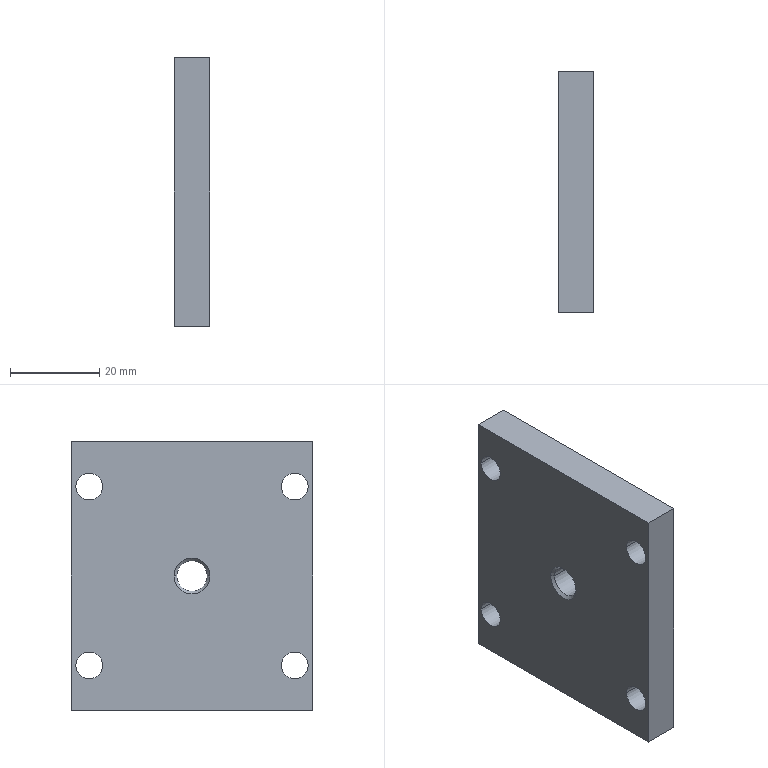Component | SolidWorks | Cover-1 | 1 solid | 18 faces | box 8 x 54 x 60 mm | volume 24720 mm3 | cylinder 10 | plane 6 | cone 2 | commonest cylinder face diameters 6 x8 6.8 x2
build123d program:
from build123d import *

# Parameters (mm, degrees)
SKETCH1_W                                            = 54
SKETCH1_H                                            = 60
BOSS_EXTRUDE1_DEPTH                                  = 8
F_6_0_6_DIAMETER_HOLE1_D                             = 6
TAPERED_COUNTERSUNK_HOLE1_FOR_M6_FLAT_HE_D           = 6.8
TAPERED_COUNTERSUNK_HOLE1_FOR_M6_FLAT_HE_CSINK_D     = 8.05
TAPERED_COUNTERSUNK_HOLE1_FOR_M6_FLAT_HE_CSINK_ANGLE = 90


with BuildPart() as part:
    # Sketch1 → Boss-Extrude1 (new body)
    with BuildSketch(Plane.XY.offset(4)):
        Rectangle(SKETCH1_W, SKETCH1_H)
    extrude(amount=-BOSS_EXTRUDE1_DEPTH)

    # 6.0 _6_ Diameter Hole1 (through all)
    with Locations(Plane(origin=(0, 0, -4), x_dir=(-1, 0, 0), z_dir=(0, 0, -1))):
        with Locations((-23, -20), (23, -20), (23, 20), (-23, 20)):
            Hole(F_6_0_6_DIAMETER_HOLE1_D / 2)

    # Tapered Countersunk Hole1 for M6 Flat He (through all)
    with Locations(Plane.XY.offset(4)):
        with Locations((0, 0)):
            CounterSinkHole(TAPERED_COUNTERSUNK_HOLE1_FOR_M6_FLAT_HE_D / 2, TAPERED_COUNTERSUNK_HOLE1_FOR_M6_FLAT_HE_CSINK_D / 2, counter_sink_angle=TAPERED_COUNTERSUNK_HOLE1_FOR_M6_FLAT_HE_CSINK_ANGLE)


solid = part.part

# Placed as in the assembly
solid = solid.moved(Location((-417, 405.75, -73.487), (90, -90, 0)))
STEP:
#1=COLOUR_RGB('',0.7922,0.8196,0.9333);
#2=FILL_AREA_STYLE_COLOUR('',#1);
#3=FILL_AREA_STYLE('',(#2));
#4=SURFACE_STYLE_FILL_AREA(#3);
#5=SURFACE_SIDE_STYLE('',(#4));
#6=SURFACE_STYLE_USAGE(.BOTH.,#5);
#7=PRESENTATION_STYLE_ASSIGNMENT((#6));
#8=CARTESIAN_POINT('',(-16.55,16.108,-2.893));
#9=VERTEX_POINT('',#8);
#10=CARTESIAN_POINT('',(-16.55,15.841,-2.893));
#11=VERTEX_POINT('',#10);
#12=CARTESIAN_POINT('',(-16.55,15.974,-2.893));
#13=DIRECTION('',(-1.,0.,-0.));
#14=DIRECTION('',(0.,-1.,0.));
#15=AXIS2_PLACEMENT_3D('',#12,#13,#14);
#16=CIRCLE('',#15,0.1339);
#17=EDGE_CURVE('',#9,#11,#16,.T.);
#18=ORIENTED_EDGE('',*,*,#17,.F.);
#19=CARTESIAN_POINT('',(-16.575,16.133,-2.893));
#20=VERTEX_POINT('',#19);
#21=CARTESIAN_POINT('',(-16.575,16.133,-2.893));
#22=DIRECTION('',(-0.7071,0.7071,0.));
#23=VECTOR('',#22,39.37);
#24=LINE('',#21,#23);
#25=EDGE_CURVE('',#9,#20,#24,.T.);
#26=ORIENTED_EDGE('',*,*,#25,.T.);
#27=CARTESIAN_POINT('',(-16.575,15.816,-2.893));
#28=VERTEX_POINT('',#27);
#29=CARTESIAN_POINT('',(-16.575,15.974,-2.893));
#30=DIRECTION('',(-1.,0.,-0.));
#31=DIRECTION('',(0.,-1.,0.));
#32=AXIS2_PLACEMENT_3D('',#29,#30,#31);
#33=CIRCLE('',#32,0.1585);
#34=EDGE_CURVE('',#20,#28,#33,.T.);
#35=ORIENTED_EDGE('',*,*,#34,.T.);
#36=CARTESIAN_POINT('',(-16.575,15.816,-2.893));
#37=DIRECTION('',(-0.7071,-0.7071,-0.));
#38=VECTOR('',#37,39.37);
#39=LINE('',#36,#38);
#40=EDGE_CURVE('',#11,#28,#39,.T.);
#41=ORIENTED_EDGE('',*,*,#40,.F.);
#42=EDGE_LOOP('',(#18,#26,#35,#41));
#43=FACE_OUTER_BOUND('',#42,.T.);
#44=CARTESIAN_POINT('',(-16.575,15.974,-2.893));
#45=DIRECTION('',(-1.,0.,-0.));
#46=DIRECTION('',(0.,-1.,0.));
#47=AXIS2_PLACEMENT_3D('',#44,#45,#46);
#48=CONICAL_SURFACE('',#47,0.1585,0.7854);
#49=ADVANCED_FACE('',(#43),#48,.F.);
#50=CARTESIAN_POINT('',(-16.26,16.108,-2.893));
#51=VERTEX_POINT('',#50);
#52=CARTESIAN_POINT('',(-16.26,15.841,-2.893));
#53=VERTEX_POINT('',#52);
#54=CARTESIAN_POINT('',(-16.26,15.974,-2.893));
#55=DIRECTION('',(-1.,0.,-0.));
#56=DIRECTION('',(0.,-1.,0.));
#57=AXIS2_PLACEMENT_3D('',#54,#55,#56);
#58=CIRCLE('',#57,0.1339);
#59=EDGE_CURVE('',#51,#53,#58,.T.);
#60=ORIENTED_EDGE('',*,*,#59,.F.);
#61=CARTESIAN_POINT('',(-16.575,16.108,-2.893));
#62=DIRECTION('',(-1.,0.,-0.));
#63=VECTOR('',#62,39.37);
#64=LINE('',#61,#63);
#65=EDGE_CURVE('',#51,#9,#64,.T.);
#66=ORIENTED_EDGE('',*,*,#65,.T.);
#67=ORIENTED_EDGE('',*,*,#17,.T.);
#68=CARTESIAN_POINT('',(-16.575,15.841,-2.893));
#69=DIRECTION('',(-1.,0.,-0.));
#70=VECTOR('',#69,39.37);
#71=LINE('',#68,#70);
#72=EDGE_CURVE('',#53,#11,#71,.T.);
#73=ORIENTED_EDGE('',*,*,#72,.F.);
#74=EDGE_LOOP('',(#60,#66,#67,#73));
#75=FACE_OUTER_BOUND('',#74,.T.);
#76=CARTESIAN_POINT('',(-16.575,15.974,-2.893));
#77=DIRECTION('',(-1.,0.,-0.));
#78=DIRECTION('',(0.,-1.,0.));
#79=AXIS2_PLACEMENT_3D('',#76,#77,#78);
#80=CYLINDRICAL_SURFACE('',#79,0.1339);
#81=ADVANCED_FACE('',(#75),#80,.F.);
#82=CARTESIAN_POINT('',(-16.575,14.951,-3.681));
#83=VERTEX_POINT('',#82);
#84=CARTESIAN_POINT('',(-16.575,15.187,-3.681));
#85=VERTEX_POINT('',#84);
#86=CARTESIAN_POINT('',(-16.575,15.069,-3.681));
#87=DIRECTION('',(1.,-0.,0.));
#88=DIRECTION('',(0.,1.,0.));
#89=AXIS2_PLACEMENT_3D('',#86,#87,#88);
#90=CIRCLE('',#89,0.1181);
#91=EDGE_CURVE('',#83,#85,#90,.T.);
#92=ORIENTED_EDGE('',*,*,#91,.F.);
#93=CARTESIAN_POINT('',(-16.26,14.951,-3.681));
#94=VERTEX_POINT('',#93);
#95=CARTESIAN_POINT('',(-16.26,14.951,-3.681));
#96=DIRECTION('',(1.,-0.,0.));
#97=VECTOR('',#96,39.37);
#98=LINE('',#95,#97);
#99=EDGE_CURVE('',#83,#94,#98,.T.);
#100=ORIENTED_EDGE('',*,*,#99,.T.);
#101=CARTESIAN_POINT('',(-16.26,15.187,-3.681));
#102=VERTEX_POINT('',#101);
#103=CARTESIAN_POINT('',(-16.26,15.069,-3.681));
#104=DIRECTION('',(1.,-0.,0.));
#105=DIRECTION('',(0.,1.,0.));
#106=AXIS2_PLACEMENT_3D('',#103,#104,#105);
#107=CIRCLE('',#106,0.1181);
#108=EDGE_CURVE('',#94,#102,#107,.T.);
#109=ORIENTED_EDGE('',*,*,#108,.T.);
#110=CARTESIAN_POINT('',(-16.26,15.187,-3.681));
#111=DIRECTION('',(1.,-0.,0.));
#112=VECTOR('',#111,39.37);
#113=LINE('',#110,#112);
#114=EDGE_CURVE('',#85,#102,#113,.T.);
#115=ORIENTED_EDGE('',*,*,#114,.F.);
#116=EDGE_LOOP('',(#92,#100,#109,#115));
#117=FACE_OUTER_BOUND('',#116,.T.);
#118=CARTESIAN_POINT('',(-16.26,15.069,-3.681));
#119=DIRECTION('',(1.,-0.,0.));
#120=DIRECTION('',(0.,1.,0.));
#121=AXIS2_PLACEMENT_3D('',#118,#119,#120);
#122=CYLINDRICAL_SURFACE('',#121,0.1181);
#123=ADVANCED_FACE('',(#117),#122,.F.);
#124=CARTESIAN_POINT('',(-16.575,16.762,-3.681));
#125=VERTEX_POINT('',#124);
#126=CARTESIAN_POINT('',(-16.575,16.998,-3.681));
#127=VERTEX_POINT('',#126);
#128=CARTESIAN_POINT('',(-16.575,16.88,-3.681));
#129=DIRECTION('',(1.,-0.,0.));
#130=DIRECTION('',(0.,1.,0.));
#131=AXIS2_PLACEMENT_3D('',#128,#129,#130);
#132=CIRCLE('',#131,0.1181);
#133=EDGE_CURVE('',#125,#127,#132,.T.);
#134=ORIENTED_EDGE('',*,*,#133,.F.);
#135=CARTESIAN_POINT('',(-16.26,16.762,-3.681));
#136=VERTEX_POINT('',#135);
#137=CARTESIAN_POINT('',(-16.26,16.762,-3.681));
#138=DIRECTION('',(1.,-0.,0.));
#139=VECTOR('',#138,39.37);
#140=LINE('',#137,#139);
#141=EDGE_CURVE('',#125,#136,#140,.T.);
#142=ORIENTED_EDGE('',*,*,#141,.T.);
#143=CARTESIAN_POINT('',(-16.26,16.998,-3.681));
#144=VERTEX_POINT('',#143);
#145=CARTESIAN_POINT('',(-16.26,16.88,-3.681));
#146=DIRECTION('',(1.,-0.,0.));
#147=DIRECTION('',(0.,1.,0.));
#148=AXIS2_PLACEMENT_3D('',#145,#146,#147);
#149=CIRCLE('',#148,0.1181);
#150=EDGE_CURVE('',#136,#144,#149,.T.);
#151=ORIENTED_EDGE('',*,*,#150,.T.);
#152=CARTESIAN_POINT('',(-16.26,16.998,-3.681));
#153=DIRECTION('',(1.,-0.,0.));
#154=VECTOR('',#153,39.37);
#155=LINE('',#152,#154);
#156=EDGE_CURVE('',#127,#144,#155,.T.);
#157=ORIENTED_EDGE('',*,*,#156,.F.);
#158=EDGE_LOOP('',(#134,#142,#151,#157));
#159=FACE_OUTER_BOUND('',#158,.T.);
#160=CARTESIAN_POINT('',(-16.26,16.88,-3.681));
#161=DIRECTION('',(1.,-0.,0.));
#162=DIRECTION('',(0.,1.,0.));
#163=AXIS2_PLACEMENT_3D('',#160,#161,#162);
#164=CYLINDRICAL_SURFACE('',#163,0.1181);
#165=ADVANCED_FACE('',(#159),#164,.F.);
#166=CARTESIAN_POINT('',(-16.575,16.762,-2.106));
#167=VERTEX_POINT('',#166);
#168=CARTESIAN_POINT('',(-16.575,16.998,-2.106));
#169=VERTEX_POINT('',#168);
#170=CARTESIAN_POINT('',(-16.575,16.88,-2.106));
#171=DIRECTION('',(1.,-0.,0.));
#172=DIRECTION('',(0.,1.,0.));
#173=AXIS2_PLACEMENT_3D('',#170,#171,#172);
#174=CIRCLE('',#173,0.1181);
#175=EDGE_CURVE('',#167,#169,#174,.T.);
#176=ORIENTED_EDGE('',*,*,#175,.F.);
#177=CARTESIAN_POINT('',(-16.26,16.762,-2.106));
#178=VERTEX_POINT('',#177);
#179=CARTESIAN_POINT('',(-16.26,16.762,-2.106));
#180=DIRECTION('',(1.,-0.,0.));
#181=VECTOR('',#180,39.37);
#182=LINE('',#179,#181);
#183=EDGE_CURVE('',#167,#178,#182,.T.);
#184=ORIENTED_EDGE('',*,*,#183,.T.);
#185=CARTESIAN_POINT('',(-16.26,16.998,-2.106));
#186=VERTEX_POINT('',#185);
#187=CARTESIAN_POINT('',(-16.26,16.88,-2.106));
#188=DIRECTION('',(1.,-0.,0.));
#189=DIRECTION('',(0.,1.,0.));
#190=AXIS2_PLACEMENT_3D('',#187,#188,#189);
#191=CIRCLE('',#190,0.1181);
#192=EDGE_CURVE('',#178,#186,#191,.T.);
#193=ORIENTED_EDGE('',*,*,#192,.T.);
#194=CARTESIAN_POINT('',(-16.26,16.998,-2.106));
#195=DIRECTION('',(1.,-0.,0.));
#196=VECTOR('',#195,39.37);
#197=LINE('',#194,#196);
#198=EDGE_CURVE('',#169,#186,#197,.T.);
#199=ORIENTED_EDGE('',*,*,#198,.F.);
#200=EDGE_LOOP('',(#176,#184,#193,#199));
#201=FACE_OUTER_BOUND('',#200,.T.);
#202=CARTESIAN_POINT('',(-16.26,16.88,-2.106));
#203=DIRECTION('',(1.,-0.,0.));
#204=DIRECTION('',(0.,1.,0.));
#205=AXIS2_PLACEMENT_3D('',#202,#203,#204);
#206=CYLINDRICAL_SURFACE('',#205,0.1181);
#207=ADVANCED_FACE('',(#201),#206,.F.);
#208=CARTESIAN_POINT('',(-16.575,14.951,-2.106));
#209=VERTEX_POINT('',#208);
#210=CARTESIAN_POINT('',(-16.575,15.187,-2.106));
#211=VERTEX_POINT('',#210);
#212=CARTESIAN_POINT('',(-16.575,15.069,-2.106));
#213=DIRECTION('',(1.,-0.,0.));
#214=DIRECTION('',(0.,1.,0.));
#215=AXIS2_PLACEMENT_3D('',#212,#213,#214);
#216=CIRCLE('',#215,0.1181);
#217=EDGE_CURVE('',#209,#211,#216,.T.);
#218=ORIENTED_EDGE('',*,*,#217,.F.);
#219=CARTESIAN_POINT('',(-16.26,14.951,-2.106));
#220=VERTEX_POINT('',#219);
#221=CARTESIAN_POINT('',(-16.26,14.951,-2.106));
#222=DIRECTION('',(1.,-0.,0.));
#223=VECTOR('',#222,39.37);
#224=LINE('',#221,#223);
#225=EDGE_CURVE('',#209,#220,#224,.T.);
#226=ORIENTED_EDGE('',*,*,#225,.T.);
#227=CARTESIAN_POINT('',(-16.26,15.187,-2.106));
#228=VERTEX_POINT('',#227);
#229=CARTESIAN_POINT('',(-16.26,15.069,-2.106));
#230=DIRECTION('',(1.,-0.,0.));
#231=DIRECTION('',(0.,1.,0.));
#232=AXIS2_PLACEMENT_3D('',#229,#230,#231);
#233=CIRCLE('',#232,0.1181);
#234=EDGE_CURVE('',#220,#228,#233,.T.);
#235=ORIENTED_EDGE('',*,*,#234,.T.);
#236=CARTESIAN_POINT('',(-16.26,15.187,-2.106));
#237=DIRECTION('',(1.,-0.,0.));
#238=VECTOR('',#237,39.37);
#239=LINE('',#236,#238);
#240=EDGE_CURVE('',#211,#228,#239,.T.);
#241=ORIENTED_EDGE('',*,*,#240,.F.);
#242=EDGE_LOOP('',(#218,#226,#235,#241));
#243=FACE_OUTER_BOUND('',#242,.T.);
#244=CARTESIAN_POINT('',(-16.26,15.069,-2.106));
#245=DIRECTION('',(1.,-0.,0.));
#246=DIRECTION('',(0.,1.,0.));
#247=AXIS2_PLACEMENT_3D('',#244,#245,#246);
#248=CYLINDRICAL_SURFACE('',#247,0.1181);
#249=ADVANCED_FACE('',(#243),#248,.F.);
#250=CARTESIAN_POINT('',(-16.575,17.037,-4.074));
#251=VERTEX_POINT('',#250);
#252=CARTESIAN_POINT('',(-16.575,14.911,-4.074));
#253=VERTEX_POINT('',#252);
#254=CARTESIAN_POINT('',(-16.575,17.037,-4.074));
#255=DIRECTION('',(-0.,-1.,-0.));
#256=VECTOR('',#255,39.37);
#257=LINE('',#254,#256);
#258=EDGE_CURVE('',#251,#253,#257,.T.);
#259=ORIENTED_EDGE('',*,*,#258,.F.);
#260=CARTESIAN_POINT('',(-16.26,17.037,-4.074));
#261=VERTEX_POINT('',#260);
#262=CARTESIAN_POINT('',(-16.26,17.037,-4.074));
#263=DIRECTION('',(-1.,0.,-0.));
#264=VECTOR('',#263,39.37);
#265=LINE('',#262,#264);
#266=EDGE_CURVE('',#261,#251,#265,.T.);
#267=ORIENTED_EDGE('',*,*,#266,.F.);
#268=CARTESIAN_POINT('',(-16.26,14.911,-4.074));
#269=VERTEX_POINT('',#268);
#270=CARTESIAN_POINT('',(-16.26,17.037,-4.074));
#271=DIRECTION('',(-0.,-1.,-0.));
#272=VECTOR('',#271,39.37);
#273=LINE('',#270,#272);
#274=EDGE_CURVE('',#261,#269,#273,.T.);
#275=ORIENTED_EDGE('',*,*,#274,.T.);
#276=CARTESIAN_POINT('',(-16.26,14.911,-4.074));
#277=DIRECTION('',(-1.,0.,-0.));
#278=VECTOR('',#277,39.37);
#279=LINE('',#276,#278);
#280=EDGE_CURVE('',#269,#253,#279,.T.);
#281=ORIENTED_EDGE('',*,*,#280,.T.);
#282=EDGE_LOOP('',(#259,#267,#275,#281));
#283=FACE_OUTER_BOUND('',#282,.T.);
#284=CARTESIAN_POINT('',(-16.26,17.037,-4.074));
#285=DIRECTION('',(0.,0.,-1.));
#286=DIRECTION('',(1.,-0.,0.));
#287=AXIS2_PLACEMENT_3D('',#284,#285,#286);
#288=PLANE('',#287);
#289=ADVANCED_FACE('',(#283),#288,.T.);
#290=CARTESIAN_POINT('',(-16.575,17.037,-1.712));
#291=VERTEX_POINT('',#290);
#292=CARTESIAN_POINT('',(-16.575,17.037,-1.712));
#293=DIRECTION('',(0.,0.,-1.));
#294=VECTOR('',#293,39.37);
#295=LINE('',#292,#294);
#296=EDGE_CURVE('',#291,#251,#295,.T.);
#297=ORIENTED_EDGE('',*,*,#296,.F.);
#298=CARTESIAN_POINT('',(-16.26,17.037,-1.712));
#299=VERTEX_POINT('',#298);
#300=CARTESIAN_POINT('',(-16.26,17.037,-1.712));
#301=DIRECTION('',(-1.,0.,-0.));
#302=VECTOR('',#301,39.37);
#303=LINE('',#300,#302);
#304=EDGE_CURVE('',#299,#291,#303,.T.);
#305=ORIENTED_EDGE('',*,*,#304,.F.);
#306=CARTESIAN_POINT('',(-16.26,17.037,-1.712));
#307=DIRECTION('',(0.,0.,-1.));
#308=VECTOR('',#307,39.37);
#309=LINE('',#306,#308);
#310=EDGE_CURVE('',#299,#261,#309,.T.);
#311=ORIENTED_EDGE('',*,*,#310,.T.);
#312=ORIENTED_EDGE('',*,*,#266,.T.);
#313=EDGE_LOOP('',(#297,#305,#311,#312));
#314=FACE_OUTER_BOUND('',#313,.T.);
#315=CARTESIAN_POINT('',(-16.26,17.037,-1.712));
#316=DIRECTION('',(0.,1.,0.));
#317=DIRECTION('',(0.,0.,-1.));
#318=AXIS2_PLACEMENT_3D('',#315,#316,#317);
#319=PLANE('',#318);
#320=ADVANCED_FACE('',(#314),#319,.T.);
#321=CARTESIAN_POINT('',(-16.575,14.911,-1.712));
#322=VERTEX_POINT('',#321);
#323=CARTESIAN_POINT('',(-16.575,14.911,-1.712));
#324=DIRECTION('',(0.,1.,0.));
#325=VECTOR('',#324,39.37);
#326=LINE('',#323,#325);
#327=EDGE_CURVE('',#322,#291,#326,.T.);
#328=ORIENTED_EDGE('',*,*,#327,.F.);
#329=CARTESIAN_POINT('',(-16.26,14.911,-1.712));
#330=VERTEX_POINT('',#329);
#331=CARTESIAN_POINT('',(-16.26,14.911,-1.712));
#332=DIRECTION('',(-1.,0.,-0.));
#333=VECTOR('',#332,39.37);
#334=LINE('',#331,#333);
#335=EDGE_CURVE('',#330,#322,#334,.T.);
#336=ORIENTED_EDGE('',*,*,#335,.F.);
#337=CARTESIAN_POINT('',(-16.26,14.911,-1.712));
#338=DIRECTION('',(0.,1.,0.));
#339=VECTOR('',#338,39.37);
#340=LINE('',#337,#339);
#341=EDGE_CURVE('',#330,#299,#340,.T.);
#342=ORIENTED_EDGE('',*,*,#341,.T.);
#343=ORIENTED_EDGE('',*,*,#304,.T.);
#344=EDGE_LOOP('',(#328,#336,#342,#343));
#345=FACE_OUTER_BOUND('',#344,.T.);
#346=CARTESIAN_POINT('',(-16.26,14.911,-1.712));
#347=DIRECTION('',(-0.,-0.,1.));
#348=DIRECTION('',(-1.,0.,-0.));
#349=AXIS2_PLACEMENT_3D('',#346,#347,#348);
#350=PLANE('',#349);
#351=ADVANCED_FACE('',(#345),#350,.T.);
#352=CARTESIAN_POINT('',(-16.575,14.911,-4.074));
#353=DIRECTION('',(-0.,-0.,1.));
#354=VECTOR('',#353,39.37);
#355=LINE('',#352,#354);
#356=EDGE_CURVE('',#253,#322,#355,.T.);
#357=ORIENTED_EDGE('',*,*,#356,.F.);
#358=ORIENTED_EDGE('',*,*,#280,.F.);
#359=CARTESIAN_POINT('',(-16.26,14.911,-4.074));
#360=DIRECTION('',(-0.,-0.,1.));
#361=VECTOR('',#360,39.37);
#362=LINE('',#359,#361);
#363=EDGE_CURVE('',#269,#330,#362,.T.);
#364=ORIENTED_EDGE('',*,*,#363,.T.);
#365=ORIENTED_EDGE('',*,*,#335,.T.);
#366=EDGE_LOOP('',(#357,#358,#364,#365));
#367=FACE_OUTER_BOUND('',#366,.T.);
#368=CARTESIAN_POINT('',(-16.26,14.911,-4.074));
#369=DIRECTION('',(-0.,-1.,-0.));
#370=DIRECTION('',(-0.,-0.,1.));
#371=AXIS2_PLACEMENT_3D('',#368,#369,#370);
#372=PLANE('',#371);
#373=ADVANCED_FACE('',(#367),#372,.T.);
#374=CARTESIAN_POINT('',(-16.26,15.974,-2.893));
#375=DIRECTION('',(-1.,0.,-0.));
#376=DIRECTION('',(0.,-1.,0.));
#377=AXIS2_PLACEMENT_3D('',#374,#375,#376);
#378=CIRCLE('',#377,0.1339);
#379=EDGE_CURVE('',#53,#51,#378,.T.);
#380=ORIENTED_EDGE('',*,*,#379,.T.);
#381=ORIENTED_EDGE('',*,*,#59,.T.);
#382=EDGE_LOOP('',(#380,#381));
#383=FACE_BOUND('',#382,.T.);
#384=CARTESIAN_POINT('',(-16.26,15.069,-3.681));
#385=DIRECTION('',(1.,-0.,0.));
#386=DIRECTION('',(0.,1.,0.));
#387=AXIS2_PLACEMENT_3D('',#384,#385,#386);
#388=CIRCLE('',#387,0.1181);
#389=EDGE_CURVE('',#102,#94,#388,.T.);
#390=ORIENTED_EDGE('',*,*,#389,.F.);
#391=ORIENTED_EDGE('',*,*,#108,.F.);
#392=EDGE_LOOP('',(#390,#391));
#393=FACE_BOUND('',#392,.T.);
#394=CARTESIAN_POINT('',(-16.26,16.88,-3.681));
#395=DIRECTION('',(1.,-0.,0.));
#396=DIRECTION('',(0.,1.,0.));
#397=AXIS2_PLACEMENT_3D('',#394,#395,#396);
#398=CIRCLE('',#397,0.1181);
#399=EDGE_CURVE('',#144,#136,#398,.T.);
#400=ORIENTED_EDGE('',*,*,#399,.F.);
#401=ORIENTED_EDGE('',*,*,#150,.F.);
#402=EDGE_LOOP('',(#400,#401));
#403=FACE_BOUND('',#402,.T.);
#404=CARTESIAN_POINT('',(-16.26,16.88,-2.106));
#405=DIRECTION('',(1.,-0.,0.));
#406=DIRECTION('',(0.,1.,0.));
#407=AXIS2_PLACEMENT_3D('',#404,#405,#406);
#408=CIRCLE('',#407,0.1181);
#409=EDGE_CURVE('',#186,#178,#408,.T.);
#410=ORIENTED_EDGE('',*,*,#409,.F.);
#411=ORIENTED_EDGE('',*,*,#192,.F.);
#412=EDGE_LOOP('',(#410,#411));
#413=FACE_BOUND('',#412,.T.);
#414=CARTESIAN_POINT('',(-16.26,15.069,-2.106));
#415=DIRECTION('',(1.,-0.,0.));
#416=DIRECTION('',(0.,1.,0.));
#417=AXIS2_PLACEMENT_3D('',#414,#415,#416);
#418=CIRCLE('',#417,0.1181);
#419=EDGE_CURVE('',#228,#220,#418,.T.);
#420=ORIENTED_EDGE('',*,*,#419,.F.);
#421=ORIENTED_EDGE('',*,*,#234,.F.);
#422=EDGE_LOOP('',(#420,#421));
#423=FACE_BOUND('',#422,.T.);
#424=ORIENTED_EDGE('',*,*,#274,.F.);
#425=ORIENTED_EDGE('',*,*,#310,.F.);
#426=ORIENTED_EDGE('',*,*,#341,.F.);
#427=ORIENTED_EDGE('',*,*,#363,.F.);
#428=EDGE_LOOP('',(#424,#425,#426,#427));
#429=FACE_OUTER_BOUND('',#428,.T.);
#430=CARTESIAN_POINT('',(-16.26,15.974,-2.893));
#431=DIRECTION('',(-1.,0.,-0.));
#432=DIRECTION('',(-0.,-1.,-0.));
#433=AXIS2_PLACEMENT_3D('',#430,#431,#432);
#434=PLANE('',#433);
#435=ADVANCED_FACE('',(#383,#393,#403,#413,#423,#429),#434,.F.);
#436=CARTESIAN_POINT('',(-16.575,15.974,-2.893));
#437=DIRECTION('',(-1.,0.,-0.));
#438=DIRECTION('',(0.,-1.,0.));
#439=AXIS2_PLACEMENT_3D('',#436,#437,#438);
#440=CIRCLE('',#439,0.1585);
#441=EDGE_CURVE('',#28,#20,#440,.T.);
#442=ORIENTED_EDGE('',*,*,#441,.F.);
#443=ORIENTED_EDGE('',*,*,#34,.F.);
#444=EDGE_LOOP('',(#442,#443));
#445=FACE_BOUND('',#444,.T.);
#446=CARTESIAN_POINT('',(-16.575,15.069,-3.681));
#447=DIRECTION('',(1.,-0.,0.));
#448=DIRECTION('',(0.,1.,0.));
#449=AXIS2_PLACEMENT_3D('',#446,#447,#448);
#450=CIRCLE('',#449,0.1181);
#451=EDGE_CURVE('',#85,#83,#450,.T.);
#452=ORIENTED_EDGE('',*,*,#451,.T.);
#453=ORIENTED_EDGE('',*,*,#91,.T.);
#454=EDGE_LOOP('',(#452,#453));
#455=FACE_BOUND('',#454,.T.);
#456=CARTESIAN_POINT('',(-16.575,16.88,-3.681));
#457=DIRECTION('',(1.,-0.,0.));
#458=DIRECTION('',(0.,1.,0.));
#459=AXIS2_PLACEMENT_3D('',#456,#457,#458);
#460=CIRCLE('',#459,0.1181);
#461=EDGE_CURVE('',#127,#125,#460,.T.);
#462=ORIENTED_EDGE('',*,*,#461,.T.);
#463=ORIENTED_EDGE('',*,*,#133,.T.);
#464=EDGE_LOOP('',(#462,#463));
#465=FACE_BOUND('',#464,.T.);
#466=CARTESIAN_POINT('',(-16.575,16.88,-2.106));
#467=DIRECTION('',(1.,-0.,0.));
#468=DIRECTION('',(0.,1.,0.));
#469=AXIS2_PLACEMENT_3D('',#466,#467,#468);
#470=CIRCLE('',#469,0.1181);
#471=EDGE_CURVE('',#169,#167,#470,.T.);
#472=ORIENTED_EDGE('',*,*,#471,.T.);
#473=ORIENTED_EDGE('',*,*,#175,.T.);
#474=EDGE_LOOP('',(#472,#473));
#475=FACE_BOUND('',#474,.T.);
#476=CARTESIAN_POINT('',(-16.575,15.069,-2.106));
#477=DIRECTION('',(1.,-0.,0.));
#478=DIRECTION('',(0.,1.,0.));
#479=AXIS2_PLACEMENT_3D('',#476,#477,#478);
#480=CIRCLE('',#479,0.1181);
#481=EDGE_CURVE('',#211,#209,#480,.T.);
#482=ORIENTED_EDGE('',*,*,#481,.T.);
#483=ORIENTED_EDGE('',*,*,#217,.T.);
#484=EDGE_LOOP('',(#482,#483));
#485=FACE_BOUND('',#484,.T.);
#486=ORIENTED_EDGE('',*,*,#258,.T.);
#487=ORIENTED_EDGE('',*,*,#356,.T.);
#488=ORIENTED_EDGE('',*,*,#327,.T.);
#489=ORIENTED_EDGE('',*,*,#296,.T.);
#490=EDGE_LOOP('',(#486,#487,#488,#489));
#491=FACE_OUTER_BOUND('',#490,.T.);
#492=CARTESIAN_POINT('',(-16.575,15.974,-2.893));
#493=DIRECTION('',(-1.,0.,-0.));
#494=DIRECTION('',(-0.,-1.,-0.));
#495=AXIS2_PLACEMENT_3D('',#492,#493,#494);
#496=PLANE('',#495);
#497=ADVANCED_FACE('',(#445,#455,#465,#475,#485,#491),#496,.T.);
#498=ORIENTED_EDGE('',*,*,#225,.F.);
#499=ORIENTED_EDGE('',*,*,#481,.F.);
#500=ORIENTED_EDGE('',*,*,#240,.T.);
#501=ORIENTED_EDGE('',*,*,#419,.T.);
#502=EDGE_LOOP('',(#498,#499,#500,#501));
#503=FACE_OUTER_BOUND('',#502,.T.);
#504=CARTESIAN_POINT('',(-16.26,15.069,-2.106));
#505=DIRECTION('',(1.,-0.,0.));
#506=DIRECTION('',(0.,1.,0.));
#507=AXIS2_PLACEMENT_3D('',#504,#505,#506);
#508=CYLINDRICAL_SURFACE('',#507,0.1181);
#509=ADVANCED_FACE('',(#503),#508,.F.);
#510=ORIENTED_EDGE('',*,*,#183,.F.);
#511=ORIENTED_EDGE('',*,*,#471,.F.);
#512=ORIENTED_EDGE('',*,*,#198,.T.);
#513=ORIENTED_EDGE('',*,*,#409,.T.);
#514=EDGE_LOOP('',(#510,#511,#512,#513));
#515=FACE_OUTER_BOUND('',#514,.T.);
#516=CARTESIAN_POINT('',(-16.26,16.88,-2.106));
#517=DIRECTION('',(1.,-0.,0.));
#518=DIRECTION('',(0.,1.,0.));
#519=AXIS2_PLACEMENT_3D('',#516,#517,#518);
#520=CYLINDRICAL_SURFACE('',#519,0.1181);
#521=ADVANCED_FACE('',(#515),#520,.F.);
#522=ORIENTED_EDGE('',*,*,#141,.F.);
#523=ORIENTED_EDGE('',*,*,#461,.F.);
#524=ORIENTED_EDGE('',*,*,#156,.T.);
#525=ORIENTED_EDGE('',*,*,#399,.T.);
#526=EDGE_LOOP('',(#522,#523,#524,#525));
#527=FACE_OUTER_BOUND('',#526,.T.);
#528=CARTESIAN_POINT('',(-16.26,16.88,-3.681));
#529=DIRECTION('',(1.,-0.,0.));
#530=DIRECTION('',(0.,1.,0.));
#531=AXIS2_PLACEMENT_3D('',#528,#529,#530);
#532=CYLINDRICAL_SURFACE('',#531,0.1181);
#533=ADVANCED_FACE('',(#527),#532,.F.);
#534=ORIENTED_EDGE('',*,*,#99,.F.);
#535=ORIENTED_EDGE('',*,*,#451,.F.);
#536=ORIENTED_EDGE('',*,*,#114,.T.);
#537=ORIENTED_EDGE('',*,*,#389,.T.);
#538=EDGE_LOOP('',(#534,#535,#536,#537));
#539=FACE_OUTER_BOUND('',#538,.T.);
#540=CARTESIAN_POINT('',(-16.26,15.069,-3.681));
#541=DIRECTION('',(1.,-0.,0.));
#542=DIRECTION('',(0.,1.,0.));
#543=AXIS2_PLACEMENT_3D('',#540,#541,#542);
#544=CYLINDRICAL_SURFACE('',#543,0.1181);
#545=ADVANCED_FACE('',(#539),#544,.F.);
#546=ORIENTED_EDGE('',*,*,#65,.F.);
#547=ORIENTED_EDGE('',*,*,#379,.F.);
#548=ORIENTED_EDGE('',*,*,#72,.T.);
#549=CARTESIAN_POINT('',(-16.55,15.974,-2.893));
#550=DIRECTION('',(-1.,0.,-0.));
#551=DIRECTION('',(0.,-1.,0.));
#552=AXIS2_PLACEMENT_3D('',#549,#550,#551);
#553=CIRCLE('',#552,0.1339);
#554=EDGE_CURVE('',#11,#9,#553,.T.);
#555=ORIENTED_EDGE('',*,*,#554,.T.);
#556=EDGE_LOOP('',(#546,#547,#548,#555));
#557=FACE_OUTER_BOUND('',#556,.T.);
#558=CARTESIAN_POINT('',(-16.575,15.974,-2.893));
#559=DIRECTION('',(-1.,0.,-0.));
#560=DIRECTION('',(0.,-1.,0.));
#561=AXIS2_PLACEMENT_3D('',#558,#559,#560);
#562=CYLINDRICAL_SURFACE('',#561,0.1339);
#563=ADVANCED_FACE('',(#557),#562,.F.);
#564=ORIENTED_EDGE('',*,*,#25,.F.);
#565=ORIENTED_EDGE('',*,*,#554,.F.);
#566=ORIENTED_EDGE('',*,*,#40,.T.);
#567=ORIENTED_EDGE('',*,*,#441,.T.);
#568=EDGE_LOOP('',(#564,#565,#566,#567));
#569=FACE_OUTER_BOUND('',#568,.T.);
#570=CARTESIAN_POINT('',(-16.575,15.974,-2.893));
#571=DIRECTION('',(-1.,0.,-0.));
#572=DIRECTION('',(0.,-1.,0.));
#573=AXIS2_PLACEMENT_3D('',#570,#571,#572);
#574=CONICAL_SURFACE('',#573,0.1585,0.7854);
#575=ADVANCED_FACE('',(#569),#574,.F.);
#576=CLOSED_SHELL('',(#49,#81,#123,#165,#207,#249,#289,#320,#351,#373,#435,#497,#509,#521,#533,#545,#563,#575));
#577=MANIFOLD_SOLID_BREP('',#576);
#578=STYLED_ITEM('',(#7),#577);
#579=PRESENTATION_LAYER_ASSIGNMENT('','',(#578));
#580=CARTESIAN_POINT('',(0.,0.,0.));
#581=DIRECTION('',(0.,0.,1.));
#582=DIRECTION('',(1.,0.,0.));
#583=AXIS2_PLACEMENT_3D('',#580,#581,#582);
#584=(LENGTH_UNIT()NAMED_UNIT(*)SI_UNIT($,.METRE.));
#585=LENGTH_MEASURE_WITH_UNIT(LENGTH_MEASURE(0.0254),#584);
#586=DIMENSIONAL_EXPONENTS(1.,0.,0.,0.,0.,0.,0.);
#587=(CONVERSION_BASED_UNIT('',#585)LENGTH_UNIT()NAMED_UNIT(#586));
#588=UNCERTAINTY_MEASURE_WITH_UNIT(LENGTH_MEASURE(0.00001),#587,'','');
#589=(NAMED_UNIT(*)PLANE_ANGLE_UNIT()SI_UNIT($,.RADIAN.));
#590=(NAMED_UNIT(*)SI_UNIT($,.STERADIAN.)SOLID_ANGLE_UNIT());
#591=(GEOMETRIC_REPRESENTATION_CONTEXT(3)GLOBAL_UNCERTAINTY_ASSIGNED_CONTEXT((#588))GLOBAL_UNIT_ASSIGNED_CONTEXT((#587,#589,#590))REPRESENTATION_CONTEXT('',''));
#592=ADVANCED_BREP_SHAPE_REPRESENTATION('',(#577,#583),#591);
#593=(LENGTH_UNIT()NAMED_UNIT(*)SI_UNIT($,.METRE.));
#594=LENGTH_MEASURE_WITH_UNIT(LENGTH_MEASURE(0.0254),#593);
#595=DIMENSIONAL_EXPONENTS(1.,0.,0.,0.,0.,0.,0.);
#596=(CONVERSION_BASED_UNIT('',#594)LENGTH_UNIT()NAMED_UNIT(#595));
#597=UNCERTAINTY_MEASURE_WITH_UNIT(LENGTH_MEASURE(0.00001),#596,'','');
#598=(NAMED_UNIT(*)PLANE_ANGLE_UNIT()SI_UNIT($,.RADIAN.));
#599=(NAMED_UNIT(*)SI_UNIT($,.STERADIAN.)SOLID_ANGLE_UNIT());
#600=(GEOMETRIC_REPRESENTATION_CONTEXT(3)GLOBAL_UNCERTAINTY_ASSIGNED_CONTEXT((#597))GLOBAL_UNIT_ASSIGNED_CONTEXT((#596,#598,#599))REPRESENTATION_CONTEXT('',''));
#601=MECHANICAL_DESIGN_GEOMETRIC_PRESENTATION_REPRESENTATION('',(#578),#600);